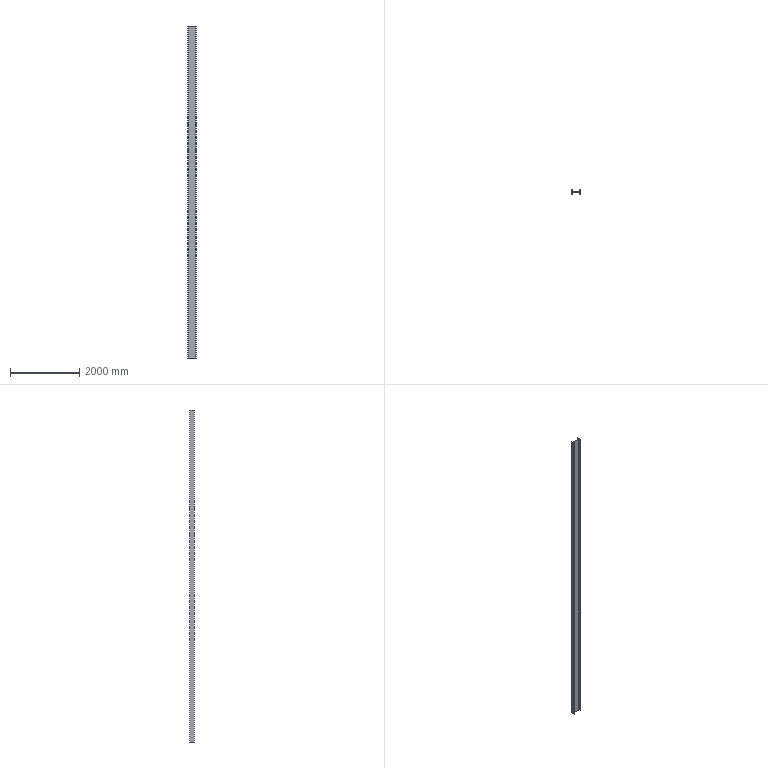Component | NX | CHUNSHUIJINCAO_DI | 1 solid | 14 faces | box 250 x 118 x 9600 mm | volume 50956800 mm3 | plane 14
STEP:
#1=CARTESIAN_POINT('',(0.,0.,0.));
#2=DIRECTION('',(0.,0.,1.));
#3=DIRECTION('',(1.,0.,0.));
#4=AXIS2_PLACEMENT_3D('',#1,#2,#3);
#5=CARTESIAN_POINT('',(2850.,6809.,250.));
#6=VERTEX_POINT('',#5);
#7=CARTESIAN_POINT('',(2850.,6691.,250.));
#8=VERTEX_POINT('',#7);
#9=CARTESIAN_POINT('',(2850.,6809.,250.));
#10=DIRECTION('',(-0.,-1.,0.));
#11=VECTOR('',#10,1.);
#12=LINE('',#9,#11);
#13=CARTESIAN_POINT('',(2850.,6809.,9850.));
#14=DIRECTION('',(1.,-0.,0.));
#15=DIRECTION('',(0.,1.,0.));
#16=AXIS2_PLACEMENT_3D('',#13,#14,#15);
#17=PLANE('',#16);
#18=CARTESIAN_POINT('',(0.,-9600.));
#19=DIRECTION('',(-1.,0.));
#20=VECTOR('',#19,1.);
#21=LINE('',#18,#20);
#22=(GEOMETRIC_REPRESENTATION_CONTEXT(2)PARAMETRIC_REPRESENTATION_CONTEXT()REPRESENTATION_CONTEXT('',''));
#23=DEFINITIONAL_REPRESENTATION('',(#21),#22);
#24=PCURVE('',#17,#23);
#25=CARTESIAN_POINT('',(2850.,6809.,250.));
#26=DIRECTION('',(0.,0.,1.));
#27=DIRECTION('',(1.,0.,0.));
#28=AXIS2_PLACEMENT_3D('',#25,#26,#27);
#29=PLANE('',#28);
#30=CARTESIAN_POINT('',(0.,0.));
#31=DIRECTION('',(-0.,-1.));
#32=VECTOR('',#31,1.);
#33=LINE('',#30,#32);
#34=(GEOMETRIC_REPRESENTATION_CONTEXT(2)PARAMETRIC_REPRESENTATION_CONTEXT()REPRESENTATION_CONTEXT('',''));
#35=DEFINITIONAL_REPRESENTATION('',(#33),#34);
#36=PCURVE('',#29,#35);
#37=SURFACE_CURVE('',#12,(#24,#36),.PCURVE_S1.);
#38=EDGE_CURVE('',#6,#8,#37,.T.);
#39=ORIENTED_EDGE('',*,*,#38,.T.);
#40=CARTESIAN_POINT('',(2850.,6691.,9850.));
#41=VERTEX_POINT('',#40);
#42=CARTESIAN_POINT('',(2850.,6691.,9850.));
#43=DIRECTION('',(0.,0.,-1.));
#44=VECTOR('',#43,1.);
#45=LINE('',#42,#44);
#46=CARTESIAN_POINT('',(-118.,0.));
#47=DIRECTION('',(0.,-1.));
#48=VECTOR('',#47,1.);
#49=LINE('',#46,#48);
#50=(GEOMETRIC_REPRESENTATION_CONTEXT(2)PARAMETRIC_REPRESENTATION_CONTEXT()REPRESENTATION_CONTEXT('',''));
#51=DEFINITIONAL_REPRESENTATION('',(#49),#50);
#52=PCURVE('',#17,#51);
#53=CARTESIAN_POINT('',(2850.,6691.,9850.));
#54=DIRECTION('',(0.,1.,0.));
#55=DIRECTION('',(0.,0.,1.));
#56=AXIS2_PLACEMENT_3D('',#53,#54,#55);
#57=PLANE('',#56);
#58=CARTESIAN_POINT('',(0.,0.));
#59=DIRECTION('',(-1.,0.));
#60=VECTOR('',#59,1.);
#61=LINE('',#58,#60);
#62=(GEOMETRIC_REPRESENTATION_CONTEXT(2)PARAMETRIC_REPRESENTATION_CONTEXT()REPRESENTATION_CONTEXT('',''));
#63=DEFINITIONAL_REPRESENTATION('',(#61),#62);
#64=PCURVE('',#57,#63);
#65=SURFACE_CURVE('',#45,(#52,#64),.PCURVE_S1.);
#66=EDGE_CURVE('',#41,#8,#65,.T.);
#67=ORIENTED_EDGE('',*,*,#66,.F.);
#68=CARTESIAN_POINT('',(2850.,6809.,9850.));
#69=VERTEX_POINT('',#68);
#70=CARTESIAN_POINT('',(2850.,6809.,9850.));
#71=DIRECTION('',(-0.,-1.,0.));
#72=VECTOR('',#71,1.);
#73=LINE('',#70,#72);
#74=CARTESIAN_POINT('',(0.,0.));
#75=DIRECTION('',(-1.,0.));
#76=VECTOR('',#75,1.);
#77=LINE('',#74,#76);
#78=(GEOMETRIC_REPRESENTATION_CONTEXT(2)PARAMETRIC_REPRESENTATION_CONTEXT()REPRESENTATION_CONTEXT('',''));
#79=DEFINITIONAL_REPRESENTATION('',(#77),#78);
#80=PCURVE('',#17,#79);
#81=CARTESIAN_POINT('',(2850.,6809.,9850.));
#82=DIRECTION('',(0.,0.,1.));
#83=DIRECTION('',(1.,0.,0.));
#84=AXIS2_PLACEMENT_3D('',#81,#82,#83);
#85=PLANE('',#84);
#86=CARTESIAN_POINT('',(0.,0.));
#87=DIRECTION('',(-0.,-1.));
#88=VECTOR('',#87,1.);
#89=LINE('',#86,#88);
#90=(GEOMETRIC_REPRESENTATION_CONTEXT(2)PARAMETRIC_REPRESENTATION_CONTEXT()REPRESENTATION_CONTEXT('',''));
#91=DEFINITIONAL_REPRESENTATION('',(#89),#90);
#92=PCURVE('',#85,#91);
#93=SURFACE_CURVE('',#73,(#80,#92),.PCURVE_S1.);
#94=EDGE_CURVE('',#69,#41,#93,.T.);
#95=ORIENTED_EDGE('',*,*,#94,.F.);
#96=CARTESIAN_POINT('',(2850.,6809.,9850.));
#97=DIRECTION('',(0.,0.,-1.));
#98=VECTOR('',#97,1.);
#99=LINE('',#96,#98);
#100=CARTESIAN_POINT('',(0.,0.));
#101=DIRECTION('',(0.,-1.));
#102=VECTOR('',#101,1.);
#103=LINE('',#100,#102);
#104=(GEOMETRIC_REPRESENTATION_CONTEXT(2)PARAMETRIC_REPRESENTATION_CONTEXT()REPRESENTATION_CONTEXT('',''));
#105=DEFINITIONAL_REPRESENTATION('',(#103),#104);
#106=PCURVE('',#17,#105);
#107=CARTESIAN_POINT('',(2863.,6809.,9850.));
#108=DIRECTION('',(0.,-1.,0.));
#109=DIRECTION('',(0.,0.,-1.));
#110=AXIS2_PLACEMENT_3D('',#107,#108,#109);
#111=PLANE('',#110);
#112=CARTESIAN_POINT('',(0.,-13.));
#113=DIRECTION('',(1.,0.));
#114=VECTOR('',#113,1.);
#115=LINE('',#112,#114);
#116=(GEOMETRIC_REPRESENTATION_CONTEXT(2)PARAMETRIC_REPRESENTATION_CONTEXT()REPRESENTATION_CONTEXT('',''));
#117=DEFINITIONAL_REPRESENTATION('',(#115),#116);
#118=PCURVE('',#111,#117);
#119=SURFACE_CURVE('',#99,(#106,#118),.PCURVE_S1.);
#120=EDGE_CURVE('',#69,#6,#119,.T.);
#121=ORIENTED_EDGE('',*,*,#120,.T.);
#122=EDGE_LOOP('',(#39,#67,#95,#121));
#123=FACE_BOUND('',#122,.T.);
#124=ADVANCED_FACE('',(#123),#17,.F.);
#125=CARTESIAN_POINT('',(2863.,6691.,250.));
#126=VERTEX_POINT('',#125);
#127=CARTESIAN_POINT('',(2850.,6691.,250.));
#128=DIRECTION('',(1.,0.,0.));
#129=VECTOR('',#128,1.);
#130=LINE('',#127,#129);
#131=CARTESIAN_POINT('',(-9600.,0.));
#132=DIRECTION('',(0.,1.));
#133=VECTOR('',#132,1.);
#134=LINE('',#131,#133);
#135=(GEOMETRIC_REPRESENTATION_CONTEXT(2)PARAMETRIC_REPRESENTATION_CONTEXT()REPRESENTATION_CONTEXT('',''));
#136=DEFINITIONAL_REPRESENTATION('',(#134),#135);
#137=PCURVE('',#57,#136);
#138=CARTESIAN_POINT('',(0.,-118.));
#139=DIRECTION('',(1.,0.));
#140=VECTOR('',#139,1.);
#141=LINE('',#138,#140);
#142=(GEOMETRIC_REPRESENTATION_CONTEXT(2)PARAMETRIC_REPRESENTATION_CONTEXT()REPRESENTATION_CONTEXT('',''));
#143=DEFINITIONAL_REPRESENTATION('',(#141),#142);
#144=PCURVE('',#29,#143);
#145=SURFACE_CURVE('',#130,(#137,#144),.PCURVE_S1.);
#146=EDGE_CURVE('',#8,#126,#145,.T.);
#147=ORIENTED_EDGE('',*,*,#146,.T.);
#148=CARTESIAN_POINT('',(2863.,6691.,9850.));
#149=VERTEX_POINT('',#148);
#150=CARTESIAN_POINT('',(2863.,6691.,9850.));
#151=DIRECTION('',(0.,0.,-1.));
#152=VECTOR('',#151,1.);
#153=LINE('',#150,#152);
#154=CARTESIAN_POINT('',(0.,13.));
#155=DIRECTION('',(-1.,0.));
#156=VECTOR('',#155,1.);
#157=LINE('',#154,#156);
#158=(GEOMETRIC_REPRESENTATION_CONTEXT(2)PARAMETRIC_REPRESENTATION_CONTEXT()REPRESENTATION_CONTEXT('',''));
#159=DEFINITIONAL_REPRESENTATION('',(#157),#158);
#160=PCURVE('',#57,#159);
#161=CARTESIAN_POINT('',(2863.,6691.,9850.));
#162=DIRECTION('',(-1.,0.,0.));
#163=DIRECTION('',(-0.,-1.,0.));
#164=AXIS2_PLACEMENT_3D('',#161,#162,#163);
#165=PLANE('',#164);
#166=CARTESIAN_POINT('',(0.,0.));
#167=DIRECTION('',(0.,-1.));
#168=VECTOR('',#167,1.);
#169=LINE('',#166,#168);
#170=(GEOMETRIC_REPRESENTATION_CONTEXT(2)PARAMETRIC_REPRESENTATION_CONTEXT()REPRESENTATION_CONTEXT('',''));
#171=DEFINITIONAL_REPRESENTATION('',(#169),#170);
#172=PCURVE('',#165,#171);
#173=SURFACE_CURVE('',#153,(#160,#172),.PCURVE_S1.);
#174=EDGE_CURVE('',#149,#126,#173,.T.);
#175=ORIENTED_EDGE('',*,*,#174,.F.);
#176=CARTESIAN_POINT('',(2850.,6691.,9850.));
#177=DIRECTION('',(1.,0.,0.));
#178=VECTOR('',#177,1.);
#179=LINE('',#176,#178);
#180=CARTESIAN_POINT('',(0.,0.));
#181=DIRECTION('',(0.,1.));
#182=VECTOR('',#181,1.);
#183=LINE('',#180,#182);
#184=(GEOMETRIC_REPRESENTATION_CONTEXT(2)PARAMETRIC_REPRESENTATION_CONTEXT()REPRESENTATION_CONTEXT('',''));
#185=DEFINITIONAL_REPRESENTATION('',(#183),#184);
#186=PCURVE('',#57,#185);
#187=CARTESIAN_POINT('',(0.,-118.));
#188=DIRECTION('',(1.,0.));
#189=VECTOR('',#188,1.);
#190=LINE('',#187,#189);
#191=(GEOMETRIC_REPRESENTATION_CONTEXT(2)PARAMETRIC_REPRESENTATION_CONTEXT()REPRESENTATION_CONTEXT('',''));
#192=DEFINITIONAL_REPRESENTATION('',(#190),#191);
#193=PCURVE('',#85,#192);
#194=SURFACE_CURVE('',#179,(#186,#193),.PCURVE_S1.);
#195=EDGE_CURVE('',#41,#149,#194,.T.);
#196=ORIENTED_EDGE('',*,*,#195,.F.);
#197=ORIENTED_EDGE('',*,*,#66,.T.);
#198=EDGE_LOOP('',(#147,#175,#196,#197));
#199=FACE_BOUND('',#198,.T.);
#200=ADVANCED_FACE('',(#199),#57,.F.);
#201=CARTESIAN_POINT('',(2863.,6745.,250.));
#202=VERTEX_POINT('',#201);
#203=CARTESIAN_POINT('',(2863.,6691.,250.));
#204=DIRECTION('',(0.,1.,0.));
#205=VECTOR('',#204,1.);
#206=LINE('',#203,#205);
#207=CARTESIAN_POINT('',(0.,-9600.));
#208=DIRECTION('',(-1.,0.));
#209=VECTOR('',#208,1.);
#210=LINE('',#207,#209);
#211=(GEOMETRIC_REPRESENTATION_CONTEXT(2)PARAMETRIC_REPRESENTATION_CONTEXT()REPRESENTATION_CONTEXT('',''));
#212=DEFINITIONAL_REPRESENTATION('',(#210),#211);
#213=PCURVE('',#165,#212);
#214=CARTESIAN_POINT('',(13.,-118.));
#215=DIRECTION('',(0.,1.));
#216=VECTOR('',#215,1.);
#217=LINE('',#214,#216);
#218=(GEOMETRIC_REPRESENTATION_CONTEXT(2)PARAMETRIC_REPRESENTATION_CONTEXT()REPRESENTATION_CONTEXT('',''));
#219=DEFINITIONAL_REPRESENTATION('',(#217),#218);
#220=PCURVE('',#29,#219);
#221=SURFACE_CURVE('',#206,(#213,#220),.PCURVE_S1.);
#222=EDGE_CURVE('',#126,#202,#221,.T.);
#223=ORIENTED_EDGE('',*,*,#222,.T.);
#224=CARTESIAN_POINT('',(2863.,6745.,9850.));
#225=VERTEX_POINT('',#224);
#226=CARTESIAN_POINT('',(2863.,6745.,9850.));
#227=DIRECTION('',(0.,0.,-1.));
#228=VECTOR('',#227,1.);
#229=LINE('',#226,#228);
#230=CARTESIAN_POINT('',(-54.,0.));
#231=DIRECTION('',(0.,-1.));
#232=VECTOR('',#231,1.);
#233=LINE('',#230,#232);
#234=(GEOMETRIC_REPRESENTATION_CONTEXT(2)PARAMETRIC_REPRESENTATION_CONTEXT()REPRESENTATION_CONTEXT('',''));
#235=DEFINITIONAL_REPRESENTATION('',(#233),#234);
#236=PCURVE('',#165,#235);
#237=CARTESIAN_POINT('',(2863.,6745.,9850.));
#238=DIRECTION('',(0.,1.,0.));
#239=DIRECTION('',(-1.,0.,0.));
#240=AXIS2_PLACEMENT_3D('',#237,#238,#239);
#241=PLANE('',#240);
#242=CARTESIAN_POINT('',(0.,0.));
#243=DIRECTION('',(0.,-1.));
#244=VECTOR('',#243,1.);
#245=LINE('',#242,#244);
#246=(GEOMETRIC_REPRESENTATION_CONTEXT(2)PARAMETRIC_REPRESENTATION_CONTEXT()REPRESENTATION_CONTEXT('',''));
#247=DEFINITIONAL_REPRESENTATION('',(#245),#246);
#248=PCURVE('',#241,#247);
#249=SURFACE_CURVE('',#229,(#236,#248),.PCURVE_S1.);
#250=EDGE_CURVE('',#225,#202,#249,.T.);
#251=ORIENTED_EDGE('',*,*,#250,.F.);
#252=CARTESIAN_POINT('',(2863.,6691.,9850.));
#253=DIRECTION('',(0.,1.,0.));
#254=VECTOR('',#253,1.);
#255=LINE('',#252,#254);
#256=CARTESIAN_POINT('',(0.,0.));
#257=DIRECTION('',(-1.,0.));
#258=VECTOR('',#257,1.);
#259=LINE('',#256,#258);
#260=(GEOMETRIC_REPRESENTATION_CONTEXT(2)PARAMETRIC_REPRESENTATION_CONTEXT()REPRESENTATION_CONTEXT('',''));
#261=DEFINITIONAL_REPRESENTATION('',(#259),#260);
#262=PCURVE('',#165,#261);
#263=CARTESIAN_POINT('',(13.,-118.));
#264=DIRECTION('',(0.,1.));
#265=VECTOR('',#264,1.);
#266=LINE('',#263,#265);
#267=(GEOMETRIC_REPRESENTATION_CONTEXT(2)PARAMETRIC_REPRESENTATION_CONTEXT()REPRESENTATION_CONTEXT('',''));
#268=DEFINITIONAL_REPRESENTATION('',(#266),#267);
#269=PCURVE('',#85,#268);
#270=SURFACE_CURVE('',#255,(#262,#269),.PCURVE_S1.);
#271=EDGE_CURVE('',#149,#225,#270,.T.);
#272=ORIENTED_EDGE('',*,*,#271,.F.);
#273=ORIENTED_EDGE('',*,*,#174,.T.);
#274=EDGE_LOOP('',(#223,#251,#272,#273));
#275=FACE_BOUND('',#274,.T.);
#276=ADVANCED_FACE('',(#275),#165,.F.);
#277=CARTESIAN_POINT('',(3087.,6745.,250.));
#278=VERTEX_POINT('',#277);
#279=CARTESIAN_POINT('',(2863.,6745.,250.));
#280=DIRECTION('',(1.,-0.,0.));
#281=VECTOR('',#280,1.);
#282=LINE('',#279,#281);
#283=CARTESIAN_POINT('',(0.,-9600.));
#284=DIRECTION('',(-1.,0.));
#285=VECTOR('',#284,1.);
#286=LINE('',#283,#285);
#287=(GEOMETRIC_REPRESENTATION_CONTEXT(2)PARAMETRIC_REPRESENTATION_CONTEXT()REPRESENTATION_CONTEXT('',''));
#288=DEFINITIONAL_REPRESENTATION('',(#286),#287);
#289=PCURVE('',#241,#288);
#290=CARTESIAN_POINT('',(13.,-64.));
#291=DIRECTION('',(1.,-0.));
#292=VECTOR('',#291,1.);
#293=LINE('',#290,#292);
#294=(GEOMETRIC_REPRESENTATION_CONTEXT(2)PARAMETRIC_REPRESENTATION_CONTEXT()REPRESENTATION_CONTEXT('',''));
#295=DEFINITIONAL_REPRESENTATION('',(#293),#294);
#296=PCURVE('',#29,#295);
#297=SURFACE_CURVE('',#282,(#289,#296),.PCURVE_S1.);
#298=EDGE_CURVE('',#202,#278,#297,.T.);
#299=ORIENTED_EDGE('',*,*,#298,.T.);
#300=CARTESIAN_POINT('',(3087.,6745.,9850.));
#301=VERTEX_POINT('',#300);
#302=CARTESIAN_POINT('',(3087.,6745.,9850.));
#303=DIRECTION('',(0.,0.,-1.));
#304=VECTOR('',#303,1.);
#305=LINE('',#302,#304);
#306=CARTESIAN_POINT('',(-224.,0.));
#307=DIRECTION('',(0.,-1.));
#308=VECTOR('',#307,1.);
#309=LINE('',#306,#308);
#310=(GEOMETRIC_REPRESENTATION_CONTEXT(2)PARAMETRIC_REPRESENTATION_CONTEXT()REPRESENTATION_CONTEXT('',''));
#311=DEFINITIONAL_REPRESENTATION('',(#309),#310);
#312=PCURVE('',#241,#311);
#313=CARTESIAN_POINT('',(3087.,6745.,9850.));
#314=DIRECTION('',(1.,-0.,0.));
#315=DIRECTION('',(0.,1.,0.));
#316=AXIS2_PLACEMENT_3D('',#313,#314,#315);
#317=PLANE('',#316);
#318=CARTESIAN_POINT('',(0.,0.));
#319=DIRECTION('',(0.,-1.));
#320=VECTOR('',#319,1.);
#321=LINE('',#318,#320);
#322=(GEOMETRIC_REPRESENTATION_CONTEXT(2)PARAMETRIC_REPRESENTATION_CONTEXT()REPRESENTATION_CONTEXT('',''));
#323=DEFINITIONAL_REPRESENTATION('',(#321),#322);
#324=PCURVE('',#317,#323);
#325=SURFACE_CURVE('',#305,(#312,#324),.PCURVE_S1.);
#326=EDGE_CURVE('',#301,#278,#325,.T.);
#327=ORIENTED_EDGE('',*,*,#326,.F.);
#328=CARTESIAN_POINT('',(2863.,6745.,9850.));
#329=DIRECTION('',(1.,-0.,0.));
#330=VECTOR('',#329,1.);
#331=LINE('',#328,#330);
#332=CARTESIAN_POINT('',(0.,0.));
#333=DIRECTION('',(-1.,0.));
#334=VECTOR('',#333,1.);
#335=LINE('',#332,#334);
#336=(GEOMETRIC_REPRESENTATION_CONTEXT(2)PARAMETRIC_REPRESENTATION_CONTEXT()REPRESENTATION_CONTEXT('',''));
#337=DEFINITIONAL_REPRESENTATION('',(#335),#336);
#338=PCURVE('',#241,#337);
#339=CARTESIAN_POINT('',(13.,-64.));
#340=DIRECTION('',(1.,-0.));
#341=VECTOR('',#340,1.);
#342=LINE('',#339,#341);
#343=(GEOMETRIC_REPRESENTATION_CONTEXT(2)PARAMETRIC_REPRESENTATION_CONTEXT()REPRESENTATION_CONTEXT('',''));
#344=DEFINITIONAL_REPRESENTATION('',(#342),#343);
#345=PCURVE('',#85,#344);
#346=SURFACE_CURVE('',#331,(#338,#345),.PCURVE_S1.);
#347=EDGE_CURVE('',#225,#301,#346,.T.);
#348=ORIENTED_EDGE('',*,*,#347,.F.);
#349=ORIENTED_EDGE('',*,*,#250,.T.);
#350=EDGE_LOOP('',(#299,#327,#348,#349));
#351=FACE_BOUND('',#350,.T.);
#352=ADVANCED_FACE('',(#351),#241,.F.);
#353=CARTESIAN_POINT('',(3087.,6691.,250.));
#354=VERTEX_POINT('',#353);
#355=CARTESIAN_POINT('',(3087.,6745.,250.));
#356=DIRECTION('',(-0.,-1.,0.));
#357=VECTOR('',#356,1.);
#358=LINE('',#355,#357);
#359=CARTESIAN_POINT('',(0.,-9600.));
#360=DIRECTION('',(-1.,0.));
#361=VECTOR('',#360,1.);
#362=LINE('',#359,#361);
#363=(GEOMETRIC_REPRESENTATION_CONTEXT(2)PARAMETRIC_REPRESENTATION_CONTEXT()REPRESENTATION_CONTEXT('',''));
#364=DEFINITIONAL_REPRESENTATION('',(#362),#363);
#365=PCURVE('',#317,#364);
#366=CARTESIAN_POINT('',(237.,-64.));
#367=DIRECTION('',(-0.,-1.));
#368=VECTOR('',#367,1.);
#369=LINE('',#366,#368);
#370=(GEOMETRIC_REPRESENTATION_CONTEXT(2)PARAMETRIC_REPRESENTATION_CONTEXT()REPRESENTATION_CONTEXT('',''));
#371=DEFINITIONAL_REPRESENTATION('',(#369),#370);
#372=PCURVE('',#29,#371);
#373=SURFACE_CURVE('',#358,(#365,#372),.PCURVE_S1.);
#374=EDGE_CURVE('',#278,#354,#373,.T.);
#375=ORIENTED_EDGE('',*,*,#374,.T.);
#376=CARTESIAN_POINT('',(3087.,6691.,9850.));
#377=VERTEX_POINT('',#376);
#378=CARTESIAN_POINT('',(3087.,6691.,9850.));
#379=DIRECTION('',(0.,0.,-1.));
#380=VECTOR('',#379,1.);
#381=LINE('',#378,#380);
#382=CARTESIAN_POINT('',(-54.,0.));
#383=DIRECTION('',(0.,-1.));
#384=VECTOR('',#383,1.);
#385=LINE('',#382,#384);
#386=(GEOMETRIC_REPRESENTATION_CONTEXT(2)PARAMETRIC_REPRESENTATION_CONTEXT()REPRESENTATION_CONTEXT('',''));
#387=DEFINITIONAL_REPRESENTATION('',(#385),#386);
#388=PCURVE('',#317,#387);
#389=CARTESIAN_POINT('',(3087.,6691.,9850.));
#390=DIRECTION('',(0.,1.,0.));
#391=DIRECTION('',(-1.,0.,0.));
#392=AXIS2_PLACEMENT_3D('',#389,#390,#391);
#393=PLANE('',#392);
#394=CARTESIAN_POINT('',(0.,0.));
#395=DIRECTION('',(0.,-1.));
#396=VECTOR('',#395,1.);
#397=LINE('',#394,#396);
#398=(GEOMETRIC_REPRESENTATION_CONTEXT(2)PARAMETRIC_REPRESENTATION_CONTEXT()REPRESENTATION_CONTEXT('',''));
#399=DEFINITIONAL_REPRESENTATION('',(#397),#398);
#400=PCURVE('',#393,#399);
#401=SURFACE_CURVE('',#381,(#388,#400),.PCURVE_S1.);
#402=EDGE_CURVE('',#377,#354,#401,.T.);
#403=ORIENTED_EDGE('',*,*,#402,.F.);
#404=CARTESIAN_POINT('',(3087.,6745.,9850.));
#405=DIRECTION('',(-0.,-1.,0.));
#406=VECTOR('',#405,1.);
#407=LINE('',#404,#406);
#408=CARTESIAN_POINT('',(0.,0.));
#409=DIRECTION('',(-1.,0.));
#410=VECTOR('',#409,1.);
#411=LINE('',#408,#410);
#412=(GEOMETRIC_REPRESENTATION_CONTEXT(2)PARAMETRIC_REPRESENTATION_CONTEXT()REPRESENTATION_CONTEXT('',''));
#413=DEFINITIONAL_REPRESENTATION('',(#411),#412);
#414=PCURVE('',#317,#413);
#415=CARTESIAN_POINT('',(237.,-64.));
#416=DIRECTION('',(-0.,-1.));
#417=VECTOR('',#416,1.);
#418=LINE('',#415,#417);
#419=(GEOMETRIC_REPRESENTATION_CONTEXT(2)PARAMETRIC_REPRESENTATION_CONTEXT()REPRESENTATION_CONTEXT('',''));
#420=DEFINITIONAL_REPRESENTATION('',(#418),#419);
#421=PCURVE('',#85,#420);
#422=SURFACE_CURVE('',#407,(#414,#421),.PCURVE_S1.);
#423=EDGE_CURVE('',#301,#377,#422,.T.);
#424=ORIENTED_EDGE('',*,*,#423,.F.);
#425=ORIENTED_EDGE('',*,*,#326,.T.);
#426=EDGE_LOOP('',(#375,#403,#424,#425));
#427=FACE_BOUND('',#426,.T.);
#428=ADVANCED_FACE('',(#427),#317,.F.);
#429=CARTESIAN_POINT('',(3100.,6691.,250.));
#430=VERTEX_POINT('',#429);
#431=CARTESIAN_POINT('',(3087.,6691.,250.));
#432=DIRECTION('',(1.,-0.,0.));
#433=VECTOR('',#432,1.);
#434=LINE('',#431,#433);
#435=CARTESIAN_POINT('',(0.,-9600.));
#436=DIRECTION('',(-1.,0.));
#437=VECTOR('',#436,1.);
#438=LINE('',#435,#437);
#439=(GEOMETRIC_REPRESENTATION_CONTEXT(2)PARAMETRIC_REPRESENTATION_CONTEXT()REPRESENTATION_CONTEXT('',''));
#440=DEFINITIONAL_REPRESENTATION('',(#438),#439);
#441=PCURVE('',#393,#440);
#442=CARTESIAN_POINT('',(237.,-118.));
#443=DIRECTION('',(1.,-0.));
#444=VECTOR('',#443,1.);
#445=LINE('',#442,#444);
#446=(GEOMETRIC_REPRESENTATION_CONTEXT(2)PARAMETRIC_REPRESENTATION_CONTEXT()REPRESENTATION_CONTEXT('',''));
#447=DEFINITIONAL_REPRESENTATION('',(#445),#446);
#448=PCURVE('',#29,#447);
#449=SURFACE_CURVE('',#434,(#441,#448),.PCURVE_S1.);
#450=EDGE_CURVE('',#354,#430,#449,.T.);
#451=ORIENTED_EDGE('',*,*,#450,.T.);
#452=CARTESIAN_POINT('',(3100.,6691.,9850.));
#453=VERTEX_POINT('',#452);
#454=CARTESIAN_POINT('',(3100.,6691.,9850.));
#455=DIRECTION('',(0.,0.,-1.));
#456=VECTOR('',#455,1.);
#457=LINE('',#454,#456);
#458=CARTESIAN_POINT('',(-13.,0.));
#459=DIRECTION('',(0.,-1.));
#460=VECTOR('',#459,1.);
#461=LINE('',#458,#460);
#462=(GEOMETRIC_REPRESENTATION_CONTEXT(2)PARAMETRIC_REPRESENTATION_CONTEXT()REPRESENTATION_CONTEXT('',''));
#463=DEFINITIONAL_REPRESENTATION('',(#461),#462);
#464=PCURVE('',#393,#463);
#465=CARTESIAN_POINT('',(3100.,6755.,9850.));
#466=DIRECTION('',(-1.,0.,0.));
#467=DIRECTION('',(-0.,-1.,0.));
#468=AXIS2_PLACEMENT_3D('',#465,#466,#467);
#469=PLANE('',#468);
#470=CARTESIAN_POINT('',(64.,0.));
#471=DIRECTION('',(0.,-1.));
#472=VECTOR('',#471,1.);
#473=LINE('',#470,#472);
#474=(GEOMETRIC_REPRESENTATION_CONTEXT(2)PARAMETRIC_REPRESENTATION_CONTEXT()REPRESENTATION_CONTEXT('',''));
#475=DEFINITIONAL_REPRESENTATION('',(#473),#474);
#476=PCURVE('',#469,#475);
#477=SURFACE_CURVE('',#457,(#464,#476),.PCURVE_S1.);
#478=EDGE_CURVE('',#453,#430,#477,.T.);
#479=ORIENTED_EDGE('',*,*,#478,.F.);
#480=CARTESIAN_POINT('',(3087.,6691.,9850.));
#481=DIRECTION('',(1.,-0.,0.));
#482=VECTOR('',#481,1.);
#483=LINE('',#480,#482);
#484=CARTESIAN_POINT('',(0.,0.));
#485=DIRECTION('',(-1.,0.));
#486=VECTOR('',#485,1.);
#487=LINE('',#484,#486);
#488=(GEOMETRIC_REPRESENTATION_CONTEXT(2)PARAMETRIC_REPRESENTATION_CONTEXT()REPRESENTATION_CONTEXT('',''));
#489=DEFINITIONAL_REPRESENTATION('',(#487),#488);
#490=PCURVE('',#393,#489);
#491=CARTESIAN_POINT('',(237.,-118.));
#492=DIRECTION('',(1.,-0.));
#493=VECTOR('',#492,1.);
#494=LINE('',#491,#493);
#495=(GEOMETRIC_REPRESENTATION_CONTEXT(2)PARAMETRIC_REPRESENTATION_CONTEXT()REPRESENTATION_CONTEXT('',''));
#496=DEFINITIONAL_REPRESENTATION('',(#494),#495);
#497=PCURVE('',#85,#496);
#498=SURFACE_CURVE('',#483,(#490,#497),.PCURVE_S1.);
#499=EDGE_CURVE('',#377,#453,#498,.T.);
#500=ORIENTED_EDGE('',*,*,#499,.F.);
#501=ORIENTED_EDGE('',*,*,#402,.T.);
#502=EDGE_LOOP('',(#451,#479,#500,#501));
#503=FACE_BOUND('',#502,.T.);
#504=ADVANCED_FACE('',(#503),#393,.F.);
#505=CARTESIAN_POINT('',(3100.,6809.,250.));
#506=VERTEX_POINT('',#505);
#507=CARTESIAN_POINT('',(3100.,6755.,250.));
#508=DIRECTION('',(0.,1.,0.));
#509=VECTOR('',#508,1.);
#510=LINE('',#507,#509);
#511=CARTESIAN_POINT('',(0.,-9600.));
#512=DIRECTION('',(-1.,0.));
#513=VECTOR('',#512,1.);
#514=LINE('',#511,#513);
#515=(GEOMETRIC_REPRESENTATION_CONTEXT(2)PARAMETRIC_REPRESENTATION_CONTEXT()REPRESENTATION_CONTEXT('',''));
#516=DEFINITIONAL_REPRESENTATION('',(#514),#515);
#517=PCURVE('',#469,#516);
#518=CARTESIAN_POINT('',(250.,-54.));
#519=DIRECTION('',(0.,1.));
#520=VECTOR('',#519,1.);
#521=LINE('',#518,#520);
#522=(GEOMETRIC_REPRESENTATION_CONTEXT(2)PARAMETRIC_REPRESENTATION_CONTEXT()REPRESENTATION_CONTEXT('',''));
#523=DEFINITIONAL_REPRESENTATION('',(#521),#522);
#524=PCURVE('',#29,#523);
#525=SURFACE_CURVE('',#510,(#517,#524),.PCURVE_S1.);
#526=EDGE_CURVE('',#430,#506,#525,.T.);
#527=ORIENTED_EDGE('',*,*,#526,.T.);
#528=CARTESIAN_POINT('',(3100.,6809.,9850.));
#529=VERTEX_POINT('',#528);
#530=CARTESIAN_POINT('',(3100.,6809.,9850.));
#531=DIRECTION('',(0.,0.,-1.));
#532=VECTOR('',#531,1.);
#533=LINE('',#530,#532);
#534=CARTESIAN_POINT('',(-54.,0.));
#535=DIRECTION('',(0.,-1.));
#536=VECTOR('',#535,1.);
#537=LINE('',#534,#536);
#538=(GEOMETRIC_REPRESENTATION_CONTEXT(2)PARAMETRIC_REPRESENTATION_CONTEXT()REPRESENTATION_CONTEXT('',''));
#539=DEFINITIONAL_REPRESENTATION('',(#537),#538);
#540=PCURVE('',#469,#539);
#541=CARTESIAN_POINT('',(3100.,6809.,9850.));
#542=DIRECTION('',(-0.,-1.,0.));
#543=DIRECTION('',(1.,-0.,0.));
#544=AXIS2_PLACEMENT_3D('',#541,#542,#543);
#545=PLANE('',#544);
#546=CARTESIAN_POINT('',(0.,0.));
#547=DIRECTION('',(0.,-1.));
#548=VECTOR('',#547,1.);
#549=LINE('',#546,#548);
#550=(GEOMETRIC_REPRESENTATION_CONTEXT(2)PARAMETRIC_REPRESENTATION_CONTEXT()REPRESENTATION_CONTEXT('',''));
#551=DEFINITIONAL_REPRESENTATION('',(#549),#550);
#552=PCURVE('',#545,#551);
#553=SURFACE_CURVE('',#533,(#540,#552),.PCURVE_S1.);
#554=EDGE_CURVE('',#529,#506,#553,.T.);
#555=ORIENTED_EDGE('',*,*,#554,.F.);
#556=CARTESIAN_POINT('',(3100.,6691.,9850.));
#557=DIRECTION('',(0.,1.,0.));
#558=VECTOR('',#557,1.);
#559=LINE('',#556,#558);
#560=CARTESIAN_POINT('',(64.,0.));
#561=DIRECTION('',(-1.,0.));
#562=VECTOR('',#561,1.);
#563=LINE('',#560,#562);
#564=(GEOMETRIC_REPRESENTATION_CONTEXT(2)PARAMETRIC_REPRESENTATION_CONTEXT()REPRESENTATION_CONTEXT('',''));
#565=DEFINITIONAL_REPRESENTATION('',(#563),#564);
#566=PCURVE('',#469,#565);
#567=CARTESIAN_POINT('',(250.,-118.));
#568=DIRECTION('',(0.,1.));
#569=VECTOR('',#568,1.);
#570=LINE('',#567,#569);
#571=(GEOMETRIC_REPRESENTATION_CONTEXT(2)PARAMETRIC_REPRESENTATION_CONTEXT()REPRESENTATION_CONTEXT('',''));
#572=DEFINITIONAL_REPRESENTATION('',(#570),#571);
#573=PCURVE('',#85,#572);
#574=SURFACE_CURVE('',#559,(#566,#573),.PCURVE_S1.);
#575=EDGE_CURVE('',#453,#529,#574,.T.);
#576=ORIENTED_EDGE('',*,*,#575,.F.);
#577=ORIENTED_EDGE('',*,*,#478,.T.);
#578=EDGE_LOOP('',(#527,#555,#576,#577));
#579=FACE_BOUND('',#578,.T.);
#580=ADVANCED_FACE('',(#579),#469,.F.);
#581=CARTESIAN_POINT('',(3087.,6809.,250.));
#582=VERTEX_POINT('',#581);
#583=CARTESIAN_POINT('',(3100.,6809.,250.));
#584=DIRECTION('',(-1.,0.,0.));
#585=VECTOR('',#584,1.);
#586=LINE('',#583,#585);
#587=CARTESIAN_POINT('',(0.,-9600.));
#588=DIRECTION('',(-1.,0.));
#589=VECTOR('',#588,1.);
#590=LINE('',#587,#589);
#591=(GEOMETRIC_REPRESENTATION_CONTEXT(2)PARAMETRIC_REPRESENTATION_CONTEXT()REPRESENTATION_CONTEXT('',''));
#592=DEFINITIONAL_REPRESENTATION('',(#590),#591);
#593=PCURVE('',#545,#592);
#594=CARTESIAN_POINT('',(250.,0.));
#595=DIRECTION('',(-1.,0.));
#596=VECTOR('',#595,1.);
#597=LINE('',#594,#596);
#598=(GEOMETRIC_REPRESENTATION_CONTEXT(2)PARAMETRIC_REPRESENTATION_CONTEXT()REPRESENTATION_CONTEXT('',''));
#599=DEFINITIONAL_REPRESENTATION('',(#597),#598);
#600=PCURVE('',#29,#599);
#601=SURFACE_CURVE('',#586,(#593,#600),.PCURVE_S1.);
#602=EDGE_CURVE('',#506,#582,#601,.T.);
#603=ORIENTED_EDGE('',*,*,#602,.T.);
#604=CARTESIAN_POINT('',(3087.,6809.,9850.));
#605=VERTEX_POINT('',#604);
#606=CARTESIAN_POINT('',(3087.,6809.,9850.));
#607=DIRECTION('',(0.,0.,-1.));
#608=VECTOR('',#607,1.);
#609=LINE('',#606,#608);
#610=CARTESIAN_POINT('',(-13.,0.));
#611=DIRECTION('',(0.,-1.));
#612=VECTOR('',#611,1.);
#613=LINE('',#610,#612);
#614=(GEOMETRIC_REPRESENTATION_CONTEXT(2)PARAMETRIC_REPRESENTATION_CONTEXT()REPRESENTATION_CONTEXT('',''));
#615=DEFINITIONAL_REPRESENTATION('',(#613),#614);
#616=PCURVE('',#545,#615);
#617=CARTESIAN_POINT('',(3087.,6809.,9850.));
#618=DIRECTION('',(1.,-0.,0.));
#619=DIRECTION('',(0.,1.,0.));
#620=AXIS2_PLACEMENT_3D('',#617,#618,#619);
#621=PLANE('',#620);
#622=CARTESIAN_POINT('',(0.,0.));
#623=DIRECTION('',(0.,-1.));
#624=VECTOR('',#623,1.);
#625=LINE('',#622,#624);
#626=(GEOMETRIC_REPRESENTATION_CONTEXT(2)PARAMETRIC_REPRESENTATION_CONTEXT()REPRESENTATION_CONTEXT('',''));
#627=DEFINITIONAL_REPRESENTATION('',(#625),#626);
#628=PCURVE('',#621,#627);
#629=SURFACE_CURVE('',#609,(#616,#628),.PCURVE_S1.);
#630=EDGE_CURVE('',#605,#582,#629,.T.);
#631=ORIENTED_EDGE('',*,*,#630,.F.);
#632=CARTESIAN_POINT('',(3100.,6809.,9850.));
#633=DIRECTION('',(-1.,0.,0.));
#634=VECTOR('',#633,1.);
#635=LINE('',#632,#634);
#636=CARTESIAN_POINT('',(0.,0.));
#637=DIRECTION('',(-1.,0.));
#638=VECTOR('',#637,1.);
#639=LINE('',#636,#638);
#640=(GEOMETRIC_REPRESENTATION_CONTEXT(2)PARAMETRIC_REPRESENTATION_CONTEXT()REPRESENTATION_CONTEXT('',''));
#641=DEFINITIONAL_REPRESENTATION('',(#639),#640);
#642=PCURVE('',#545,#641);
#643=CARTESIAN_POINT('',(250.,0.));
#644=DIRECTION('',(-1.,0.));
#645=VECTOR('',#644,1.);
#646=LINE('',#643,#645);
#647=(GEOMETRIC_REPRESENTATION_CONTEXT(2)PARAMETRIC_REPRESENTATION_CONTEXT()REPRESENTATION_CONTEXT('',''));
#648=DEFINITIONAL_REPRESENTATION('',(#646),#647);
#649=PCURVE('',#85,#648);
#650=SURFACE_CURVE('',#635,(#642,#649),.PCURVE_S1.);
#651=EDGE_CURVE('',#529,#605,#650,.T.);
#652=ORIENTED_EDGE('',*,*,#651,.F.);
#653=ORIENTED_EDGE('',*,*,#554,.T.);
#654=EDGE_LOOP('',(#603,#631,#652,#653));
#655=FACE_BOUND('',#654,.T.);
#656=ADVANCED_FACE('',(#655),#545,.F.);
#657=CARTESIAN_POINT('',(3087.,6755.,250.));
#658=VERTEX_POINT('',#657);
#659=CARTESIAN_POINT('',(3087.,6809.,250.));
#660=DIRECTION('',(-0.,-1.,0.));
#661=VECTOR('',#660,1.);
#662=LINE('',#659,#661);
#663=CARTESIAN_POINT('',(0.,-9600.));
#664=DIRECTION('',(-1.,0.));
#665=VECTOR('',#664,1.);
#666=LINE('',#663,#665);
#667=(GEOMETRIC_REPRESENTATION_CONTEXT(2)PARAMETRIC_REPRESENTATION_CONTEXT()REPRESENTATION_CONTEXT('',''));
#668=DEFINITIONAL_REPRESENTATION('',(#666),#667);
#669=PCURVE('',#621,#668);
#670=CARTESIAN_POINT('',(237.,0.));
#671=DIRECTION('',(-0.,-1.));
#672=VECTOR('',#671,1.);
#673=LINE('',#670,#672);
#674=(GEOMETRIC_REPRESENTATION_CONTEXT(2)PARAMETRIC_REPRESENTATION_CONTEXT()REPRESENTATION_CONTEXT('',''));
#675=DEFINITIONAL_REPRESENTATION('',(#673),#674);
#676=PCURVE('',#29,#675);
#677=SURFACE_CURVE('',#662,(#669,#676),.PCURVE_S1.);
#678=EDGE_CURVE('',#582,#658,#677,.T.);
#679=ORIENTED_EDGE('',*,*,#678,.T.);
#680=CARTESIAN_POINT('',(3087.,6755.,9850.));
#681=VERTEX_POINT('',#680);
#682=CARTESIAN_POINT('',(3087.,6755.,9850.));
#683=DIRECTION('',(0.,0.,-1.));
#684=VECTOR('',#683,1.);
#685=LINE('',#682,#684);
#686=CARTESIAN_POINT('',(-54.,0.));
#687=DIRECTION('',(0.,-1.));
#688=VECTOR('',#687,1.);
#689=LINE('',#686,#688);
#690=(GEOMETRIC_REPRESENTATION_CONTEXT(2)PARAMETRIC_REPRESENTATION_CONTEXT()REPRESENTATION_CONTEXT('',''));
#691=DEFINITIONAL_REPRESENTATION('',(#689),#690);
#692=PCURVE('',#621,#691);
#693=CARTESIAN_POINT('',(3087.,6755.,9850.));
#694=DIRECTION('',(-0.,-1.,0.));
#695=DIRECTION('',(1.,-0.,0.));
#696=AXIS2_PLACEMENT_3D('',#693,#694,#695);
#697=PLANE('',#696);
#698=CARTESIAN_POINT('',(0.,0.));
#699=DIRECTION('',(0.,-1.));
#700=VECTOR('',#699,1.);
#701=LINE('',#698,#700);
#702=(GEOMETRIC_REPRESENTATION_CONTEXT(2)PARAMETRIC_REPRESENTATION_CONTEXT()REPRESENTATION_CONTEXT('',''));
#703=DEFINITIONAL_REPRESENTATION('',(#701),#702);
#704=PCURVE('',#697,#703);
#705=SURFACE_CURVE('',#685,(#692,#704),.PCURVE_S1.);
#706=EDGE_CURVE('',#681,#658,#705,.T.);
#707=ORIENTED_EDGE('',*,*,#706,.F.);
#708=CARTESIAN_POINT('',(3087.,6809.,9850.));
#709=DIRECTION('',(-0.,-1.,0.));
#710=VECTOR('',#709,1.);
#711=LINE('',#708,#710);
#712=CARTESIAN_POINT('',(0.,0.));
#713=DIRECTION('',(-1.,0.));
#714=VECTOR('',#713,1.);
#715=LINE('',#712,#714);
#716=(GEOMETRIC_REPRESENTATION_CONTEXT(2)PARAMETRIC_REPRESENTATION_CONTEXT()REPRESENTATION_CONTEXT('',''));
#717=DEFINITIONAL_REPRESENTATION('',(#715),#716);
#718=PCURVE('',#621,#717);
#719=CARTESIAN_POINT('',(237.,0.));
#720=DIRECTION('',(-0.,-1.));
#721=VECTOR('',#720,1.);
#722=LINE('',#719,#721);
#723=(GEOMETRIC_REPRESENTATION_CONTEXT(2)PARAMETRIC_REPRESENTATION_CONTEXT()REPRESENTATION_CONTEXT('',''));
#724=DEFINITIONAL_REPRESENTATION('',(#722),#723);
#725=PCURVE('',#85,#724);
#726=SURFACE_CURVE('',#711,(#718,#725),.PCURVE_S1.);
#727=EDGE_CURVE('',#605,#681,#726,.T.);
#728=ORIENTED_EDGE('',*,*,#727,.F.);
#729=ORIENTED_EDGE('',*,*,#630,.T.);
#730=EDGE_LOOP('',(#679,#707,#728,#729));
#731=FACE_BOUND('',#730,.T.);
#732=ADVANCED_FACE('',(#731),#621,.F.);
#733=CARTESIAN_POINT('',(2863.,6755.,250.));
#734=VERTEX_POINT('',#733);
#735=CARTESIAN_POINT('',(3087.,6755.,250.));
#736=DIRECTION('',(-1.,0.,0.));
#737=VECTOR('',#736,1.);
#738=LINE('',#735,#737);
#739=CARTESIAN_POINT('',(0.,-9600.));
#740=DIRECTION('',(-1.,0.));
#741=VECTOR('',#740,1.);
#742=LINE('',#739,#741);
#743=(GEOMETRIC_REPRESENTATION_CONTEXT(2)PARAMETRIC_REPRESENTATION_CONTEXT()REPRESENTATION_CONTEXT('',''));
#744=DEFINITIONAL_REPRESENTATION('',(#742),#743);
#745=PCURVE('',#697,#744);
#746=CARTESIAN_POINT('',(237.,-54.));
#747=DIRECTION('',(-1.,0.));
#748=VECTOR('',#747,1.);
#749=LINE('',#746,#748);
#750=(GEOMETRIC_REPRESENTATION_CONTEXT(2)PARAMETRIC_REPRESENTATION_CONTEXT()REPRESENTATION_CONTEXT('',''));
#751=DEFINITIONAL_REPRESENTATION('',(#749),#750);
#752=PCURVE('',#29,#751);
#753=SURFACE_CURVE('',#738,(#745,#752),.PCURVE_S1.);
#754=EDGE_CURVE('',#658,#734,#753,.T.);
#755=ORIENTED_EDGE('',*,*,#754,.T.);
#756=CARTESIAN_POINT('',(2863.,6755.,9850.));
#757=VERTEX_POINT('',#756);
#758=CARTESIAN_POINT('',(2863.,6755.,9850.));
#759=DIRECTION('',(0.,0.,-1.));
#760=VECTOR('',#759,1.);
#761=LINE('',#758,#760);
#762=CARTESIAN_POINT('',(-224.,0.));
#763=DIRECTION('',(0.,-1.));
#764=VECTOR('',#763,1.);
#765=LINE('',#762,#764);
#766=(GEOMETRIC_REPRESENTATION_CONTEXT(2)PARAMETRIC_REPRESENTATION_CONTEXT()REPRESENTATION_CONTEXT('',''));
#767=DEFINITIONAL_REPRESENTATION('',(#765),#766);
#768=PCURVE('',#697,#767);
#769=CARTESIAN_POINT('',(2863.,6755.,9850.));
#770=DIRECTION('',(-1.,0.,0.));
#771=DIRECTION('',(-0.,-1.,0.));
#772=AXIS2_PLACEMENT_3D('',#769,#770,#771);
#773=PLANE('',#772);
#774=CARTESIAN_POINT('',(0.,0.));
#775=DIRECTION('',(0.,-1.));
#776=VECTOR('',#775,1.);
#777=LINE('',#774,#776);
#778=(GEOMETRIC_REPRESENTATION_CONTEXT(2)PARAMETRIC_REPRESENTATION_CONTEXT()REPRESENTATION_CONTEXT('',''));
#779=DEFINITIONAL_REPRESENTATION('',(#777),#778);
#780=PCURVE('',#773,#779);
#781=SURFACE_CURVE('',#761,(#768,#780),.PCURVE_S1.);
#782=EDGE_CURVE('',#757,#734,#781,.T.);
#783=ORIENTED_EDGE('',*,*,#782,.F.);
#784=CARTESIAN_POINT('',(3087.,6755.,9850.));
#785=DIRECTION('',(-1.,0.,0.));
#786=VECTOR('',#785,1.);
#787=LINE('',#784,#786);
#788=CARTESIAN_POINT('',(0.,0.));
#789=DIRECTION('',(-1.,0.));
#790=VECTOR('',#789,1.);
#791=LINE('',#788,#790);
#792=(GEOMETRIC_REPRESENTATION_CONTEXT(2)PARAMETRIC_REPRESENTATION_CONTEXT()REPRESENTATION_CONTEXT('',''));
#793=DEFINITIONAL_REPRESENTATION('',(#791),#792);
#794=PCURVE('',#697,#793);
#795=CARTESIAN_POINT('',(237.,-54.));
#796=DIRECTION('',(-1.,0.));
#797=VECTOR('',#796,1.);
#798=LINE('',#795,#797);
#799=(GEOMETRIC_REPRESENTATION_CONTEXT(2)PARAMETRIC_REPRESENTATION_CONTEXT()REPRESENTATION_CONTEXT('',''));
#800=DEFINITIONAL_REPRESENTATION('',(#798),#799);
#801=PCURVE('',#85,#800);
#802=SURFACE_CURVE('',#787,(#794,#801),.PCURVE_S1.);
#803=EDGE_CURVE('',#681,#757,#802,.T.);
#804=ORIENTED_EDGE('',*,*,#803,.F.);
#805=ORIENTED_EDGE('',*,*,#706,.T.);
#806=EDGE_LOOP('',(#755,#783,#804,#805));
#807=FACE_BOUND('',#806,.T.);
#808=ADVANCED_FACE('',(#807),#697,.F.);
#809=CARTESIAN_POINT('',(2863.,6809.,250.));
#810=VERTEX_POINT('',#809);
#811=CARTESIAN_POINT('',(2863.,6755.,250.));
#812=DIRECTION('',(0.,1.,0.));
#813=VECTOR('',#812,1.);
#814=LINE('',#811,#813);
#815=CARTESIAN_POINT('',(0.,-9600.));
#816=DIRECTION('',(-1.,0.));
#817=VECTOR('',#816,1.);
#818=LINE('',#815,#817);
#819=(GEOMETRIC_REPRESENTATION_CONTEXT(2)PARAMETRIC_REPRESENTATION_CONTEXT()REPRESENTATION_CONTEXT('',''));
#820=DEFINITIONAL_REPRESENTATION('',(#818),#819);
#821=PCURVE('',#773,#820);
#822=CARTESIAN_POINT('',(13.,-54.));
#823=DIRECTION('',(0.,1.));
#824=VECTOR('',#823,1.);
#825=LINE('',#822,#824);
#826=(GEOMETRIC_REPRESENTATION_CONTEXT(2)PARAMETRIC_REPRESENTATION_CONTEXT()REPRESENTATION_CONTEXT('',''));
#827=DEFINITIONAL_REPRESENTATION('',(#825),#826);
#828=PCURVE('',#29,#827);
#829=SURFACE_CURVE('',#814,(#821,#828),.PCURVE_S1.);
#830=EDGE_CURVE('',#734,#810,#829,.T.);
#831=ORIENTED_EDGE('',*,*,#830,.T.);
#832=CARTESIAN_POINT('',(2863.,6809.,9850.));
#833=VERTEX_POINT('',#832);
#834=CARTESIAN_POINT('',(2863.,6809.,9850.));
#835=DIRECTION('',(0.,0.,-1.));
#836=VECTOR('',#835,1.);
#837=LINE('',#834,#836);
#838=CARTESIAN_POINT('',(-54.,0.));
#839=DIRECTION('',(0.,-1.));
#840=VECTOR('',#839,1.);
#841=LINE('',#838,#840);
#842=(GEOMETRIC_REPRESENTATION_CONTEXT(2)PARAMETRIC_REPRESENTATION_CONTEXT()REPRESENTATION_CONTEXT('',''));
#843=DEFINITIONAL_REPRESENTATION('',(#841),#842);
#844=PCURVE('',#773,#843);
#845=CARTESIAN_POINT('',(0.,0.));
#846=DIRECTION('',(1.,0.));
#847=VECTOR('',#846,1.);
#848=LINE('',#845,#847);
#849=(GEOMETRIC_REPRESENTATION_CONTEXT(2)PARAMETRIC_REPRESENTATION_CONTEXT()REPRESENTATION_CONTEXT('',''));
#850=DEFINITIONAL_REPRESENTATION('',(#848),#849);
#851=PCURVE('',#111,#850);
#852=SURFACE_CURVE('',#837,(#844,#851),.PCURVE_S1.);
#853=EDGE_CURVE('',#833,#810,#852,.T.);
#854=ORIENTED_EDGE('',*,*,#853,.F.);
#855=CARTESIAN_POINT('',(2863.,6755.,9850.));
#856=DIRECTION('',(0.,1.,0.));
#857=VECTOR('',#856,1.);
#858=LINE('',#855,#857);
#859=CARTESIAN_POINT('',(0.,0.));
#860=DIRECTION('',(-1.,0.));
#861=VECTOR('',#860,1.);
#862=LINE('',#859,#861);
#863=(GEOMETRIC_REPRESENTATION_CONTEXT(2)PARAMETRIC_REPRESENTATION_CONTEXT()REPRESENTATION_CONTEXT('',''));
#864=DEFINITIONAL_REPRESENTATION('',(#862),#863);
#865=PCURVE('',#773,#864);
#866=CARTESIAN_POINT('',(13.,-54.));
#867=DIRECTION('',(0.,1.));
#868=VECTOR('',#867,1.);
#869=LINE('',#866,#868);
#870=(GEOMETRIC_REPRESENTATION_CONTEXT(2)PARAMETRIC_REPRESENTATION_CONTEXT()REPRESENTATION_CONTEXT('',''));
#871=DEFINITIONAL_REPRESENTATION('',(#869),#870);
#872=PCURVE('',#85,#871);
#873=SURFACE_CURVE('',#858,(#865,#872),.PCURVE_S1.);
#874=EDGE_CURVE('',#757,#833,#873,.T.);
#875=ORIENTED_EDGE('',*,*,#874,.F.);
#876=ORIENTED_EDGE('',*,*,#782,.T.);
#877=EDGE_LOOP('',(#831,#854,#875,#876));
#878=FACE_BOUND('',#877,.T.);
#879=ADVANCED_FACE('',(#878),#773,.F.);
#880=CARTESIAN_POINT('',(2863.,6809.,250.));
#881=DIRECTION('',(-1.,0.,0.));
#882=VECTOR('',#881,1.);
#883=LINE('',#880,#882);
#884=CARTESIAN_POINT('',(9600.,0.));
#885=DIRECTION('',(0.,-1.));
#886=VECTOR('',#885,1.);
#887=LINE('',#884,#886);
#888=(GEOMETRIC_REPRESENTATION_CONTEXT(2)PARAMETRIC_REPRESENTATION_CONTEXT()REPRESENTATION_CONTEXT('',''));
#889=DEFINITIONAL_REPRESENTATION('',(#887),#888);
#890=PCURVE('',#111,#889);
#891=CARTESIAN_POINT('',(13.,0.));
#892=DIRECTION('',(-1.,0.));
#893=VECTOR('',#892,1.);
#894=LINE('',#891,#893);
#895=(GEOMETRIC_REPRESENTATION_CONTEXT(2)PARAMETRIC_REPRESENTATION_CONTEXT()REPRESENTATION_CONTEXT('',''));
#896=DEFINITIONAL_REPRESENTATION('',(#894),#895);
#897=PCURVE('',#29,#896);
#898=SURFACE_CURVE('',#883,(#890,#897),.PCURVE_S1.);
#899=EDGE_CURVE('',#810,#6,#898,.T.);
#900=ORIENTED_EDGE('',*,*,#899,.T.);
#901=ORIENTED_EDGE('',*,*,#120,.F.);
#902=CARTESIAN_POINT('',(2863.,6809.,9850.));
#903=DIRECTION('',(-1.,0.,0.));
#904=VECTOR('',#903,1.);
#905=LINE('',#902,#904);
#906=CARTESIAN_POINT('',(0.,0.));
#907=DIRECTION('',(0.,-1.));
#908=VECTOR('',#907,1.);
#909=LINE('',#906,#908);
#910=(GEOMETRIC_REPRESENTATION_CONTEXT(2)PARAMETRIC_REPRESENTATION_CONTEXT()REPRESENTATION_CONTEXT('',''));
#911=DEFINITIONAL_REPRESENTATION('',(#909),#910);
#912=PCURVE('',#111,#911);
#913=CARTESIAN_POINT('',(13.,0.));
#914=DIRECTION('',(-1.,0.));
#915=VECTOR('',#914,1.);
#916=LINE('',#913,#915);
#917=(GEOMETRIC_REPRESENTATION_CONTEXT(2)PARAMETRIC_REPRESENTATION_CONTEXT()REPRESENTATION_CONTEXT('',''));
#918=DEFINITIONAL_REPRESENTATION('',(#916),#917);
#919=PCURVE('',#85,#918);
#920=SURFACE_CURVE('',#905,(#912,#919),.PCURVE_S1.);
#921=EDGE_CURVE('',#833,#69,#920,.T.);
#922=ORIENTED_EDGE('',*,*,#921,.F.);
#923=ORIENTED_EDGE('',*,*,#853,.T.);
#924=EDGE_LOOP('',(#900,#901,#922,#923));
#925=FACE_BOUND('',#924,.T.);
#926=ADVANCED_FACE('',(#925),#111,.F.);
#927=ORIENTED_EDGE('',*,*,#94,.T.);
#928=ORIENTED_EDGE('',*,*,#195,.T.);
#929=ORIENTED_EDGE('',*,*,#271,.T.);
#930=ORIENTED_EDGE('',*,*,#347,.T.);
#931=ORIENTED_EDGE('',*,*,#423,.T.);
#932=ORIENTED_EDGE('',*,*,#499,.T.);
#933=ORIENTED_EDGE('',*,*,#575,.T.);
#934=ORIENTED_EDGE('',*,*,#651,.T.);
#935=ORIENTED_EDGE('',*,*,#727,.T.);
#936=ORIENTED_EDGE('',*,*,#803,.T.);
#937=ORIENTED_EDGE('',*,*,#874,.T.);
#938=ORIENTED_EDGE('',*,*,#921,.T.);
#939=EDGE_LOOP('',(#927,#928,#929,#930,#931,#932,#933,#934,#935,#936,#937,#938));
#940=FACE_BOUND('',#939,.T.);
#941=ADVANCED_FACE('',(#940),#85,.T.);
#942=ORIENTED_EDGE('',*,*,#38,.F.);
#943=ORIENTED_EDGE('',*,*,#899,.F.);
#944=ORIENTED_EDGE('',*,*,#830,.F.);
#945=ORIENTED_EDGE('',*,*,#754,.F.);
#946=ORIENTED_EDGE('',*,*,#678,.F.);
#947=ORIENTED_EDGE('',*,*,#602,.F.);
#948=ORIENTED_EDGE('',*,*,#526,.F.);
#949=ORIENTED_EDGE('',*,*,#450,.F.);
#950=ORIENTED_EDGE('',*,*,#374,.F.);
#951=ORIENTED_EDGE('',*,*,#298,.F.);
#952=ORIENTED_EDGE('',*,*,#222,.F.);
#953=ORIENTED_EDGE('',*,*,#146,.F.);
#954=EDGE_LOOP('',(#942,#943,#944,#945,#946,#947,#948,#949,#950,#951,#952,#953));
#955=FACE_BOUND('',#954,.T.);
#956=ADVANCED_FACE('',(#955),#29,.F.);
#957=CLOSED_SHELL('',(#124,#200,#276,#352,#428,#504,#580,#656,#732,#808,#879,#926,#941,#956));
#958=MANIFOLD_SOLID_BREP('',#957);
#959=(LENGTH_UNIT()NAMED_UNIT(*)SI_UNIT(.MILLI.,.METRE.));
#960=UNCERTAINTY_MEASURE_WITH_UNIT(LENGTH_MEASURE(0.0000001),#959,'','');
#961=(NAMED_UNIT(*)PLANE_ANGLE_UNIT()SI_UNIT($,.RADIAN.));
#962=(NAMED_UNIT(*)SI_UNIT($,.STERADIAN.)SOLID_ANGLE_UNIT());
#963=(GEOMETRIC_REPRESENTATION_CONTEXT(3)GLOBAL_UNCERTAINTY_ASSIGNED_CONTEXT((#960))GLOBAL_UNIT_ASSIGNED_CONTEXT((#959,#961,#962))REPRESENTATION_CONTEXT('',''));
#964=ADVANCED_BREP_SHAPE_REPRESENTATION('',(#4,#958),#963);